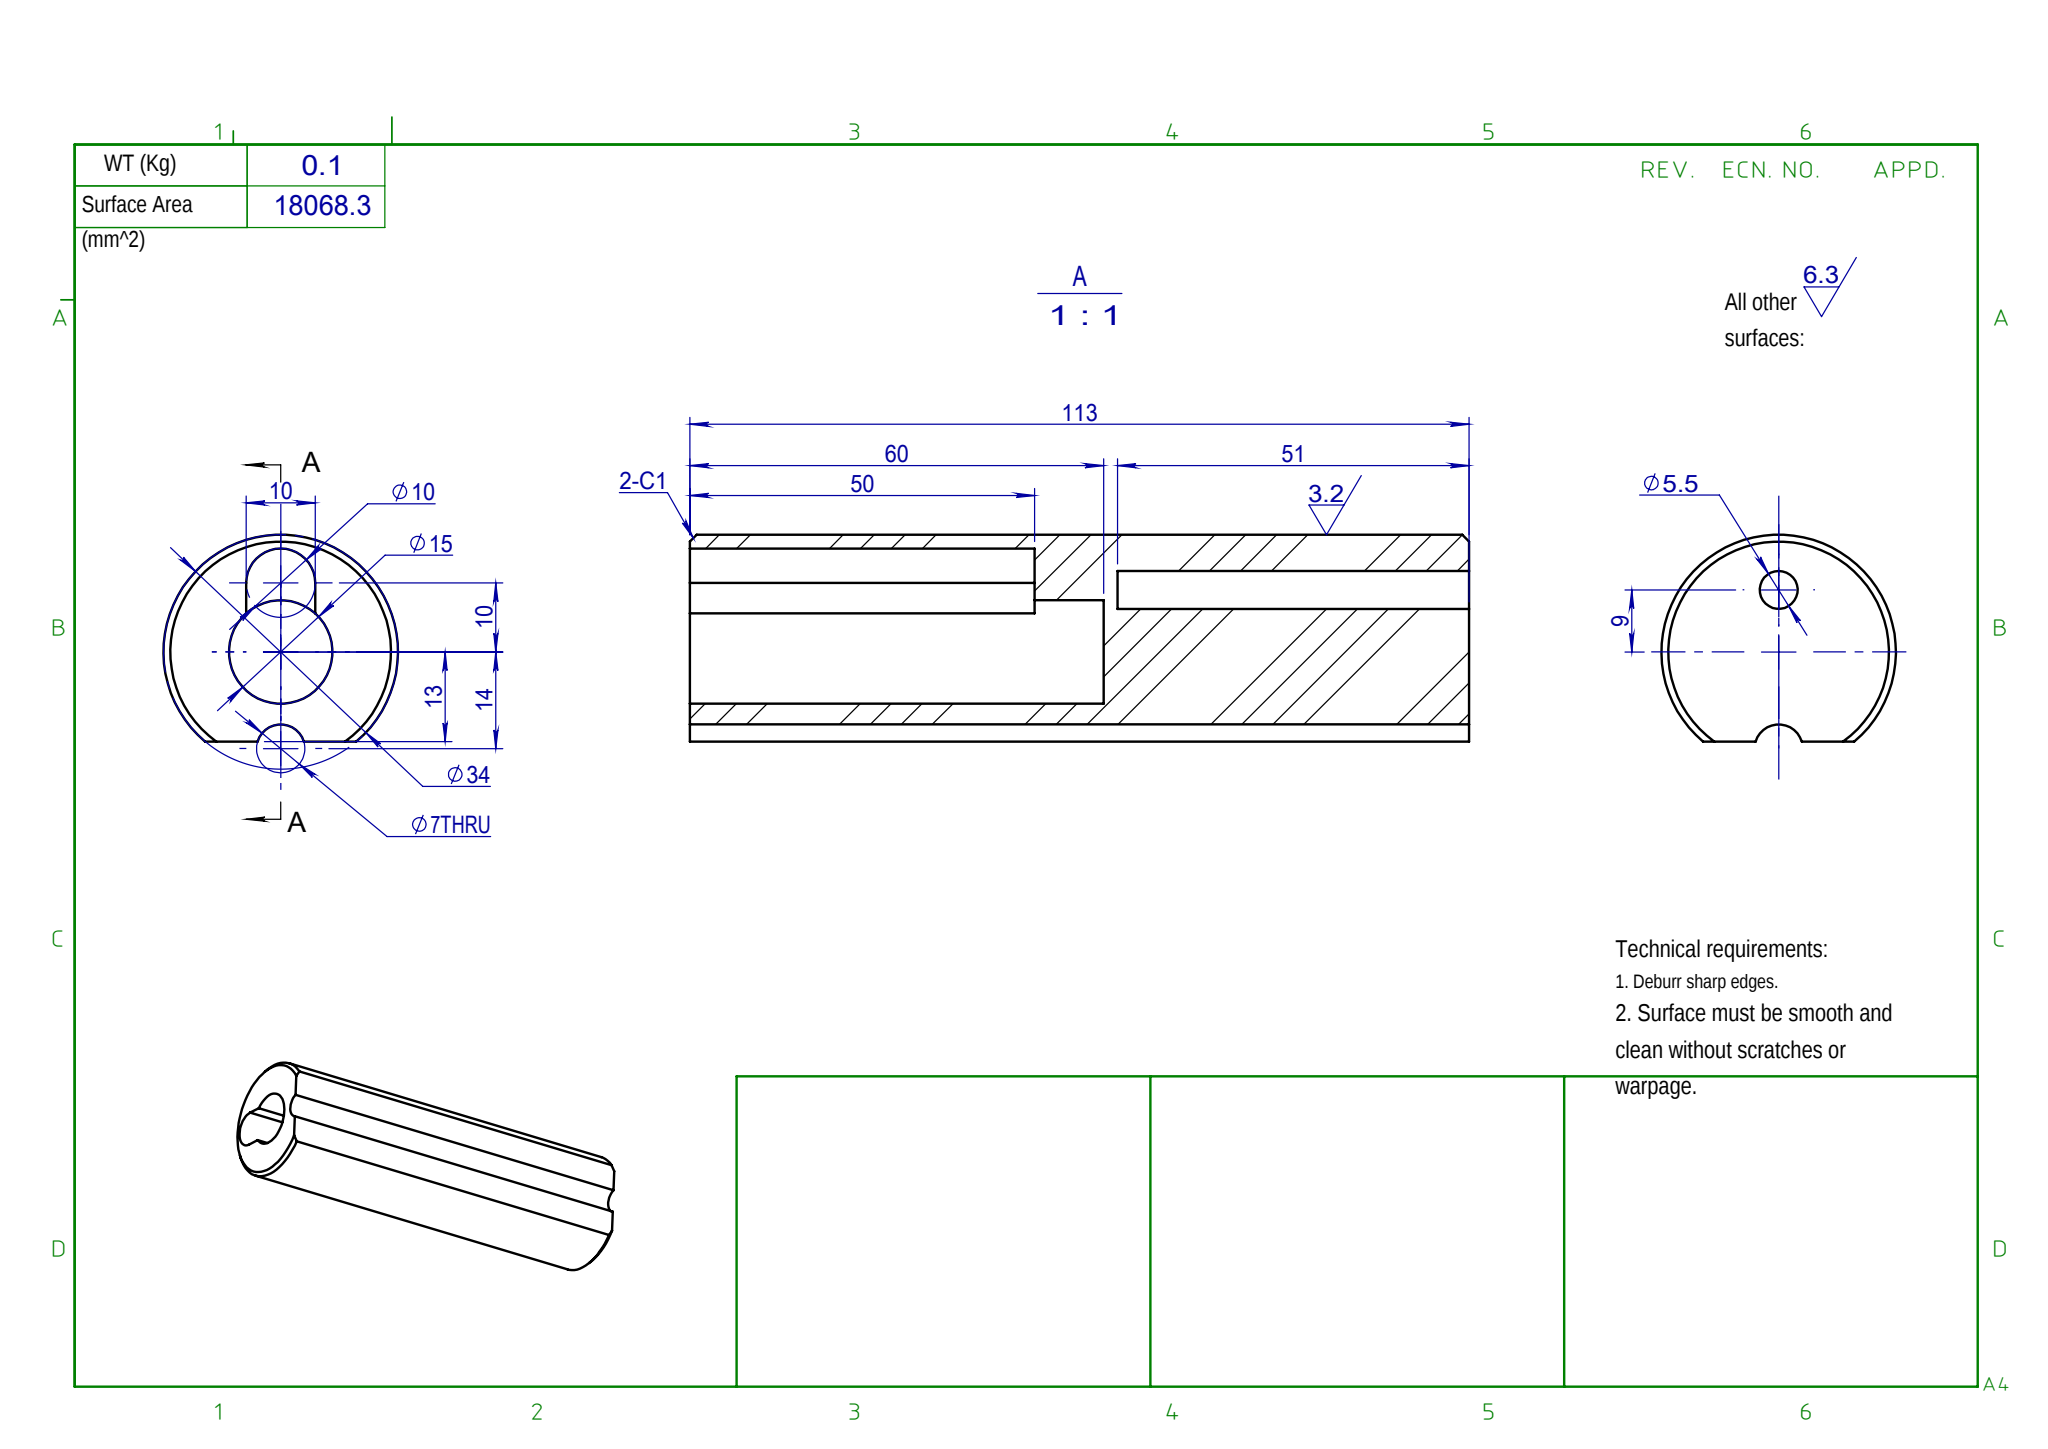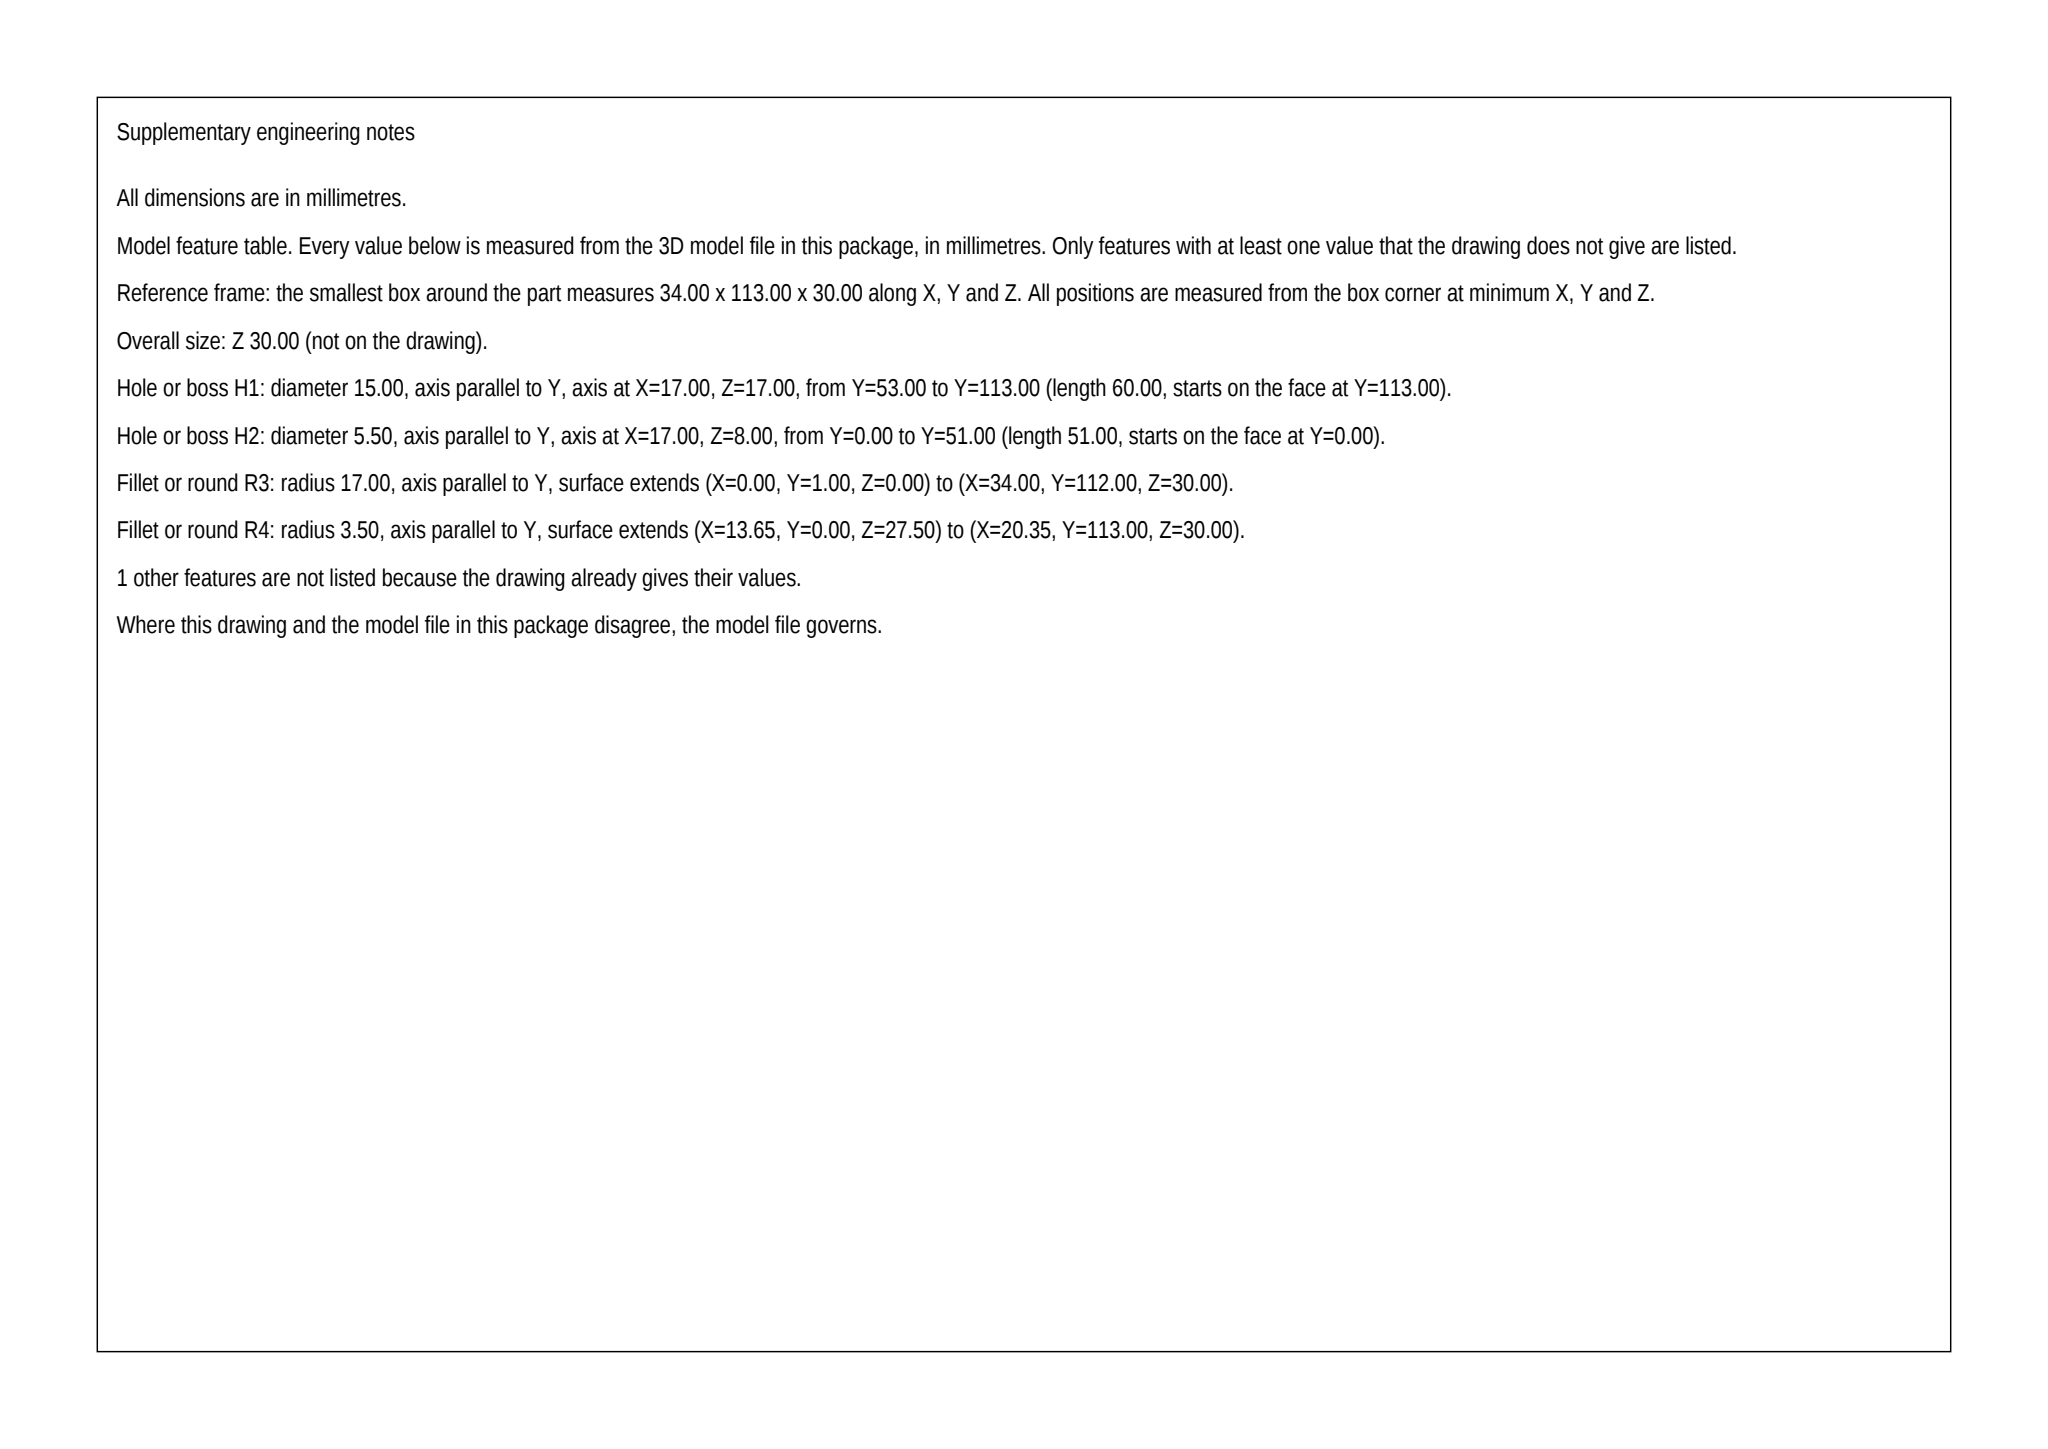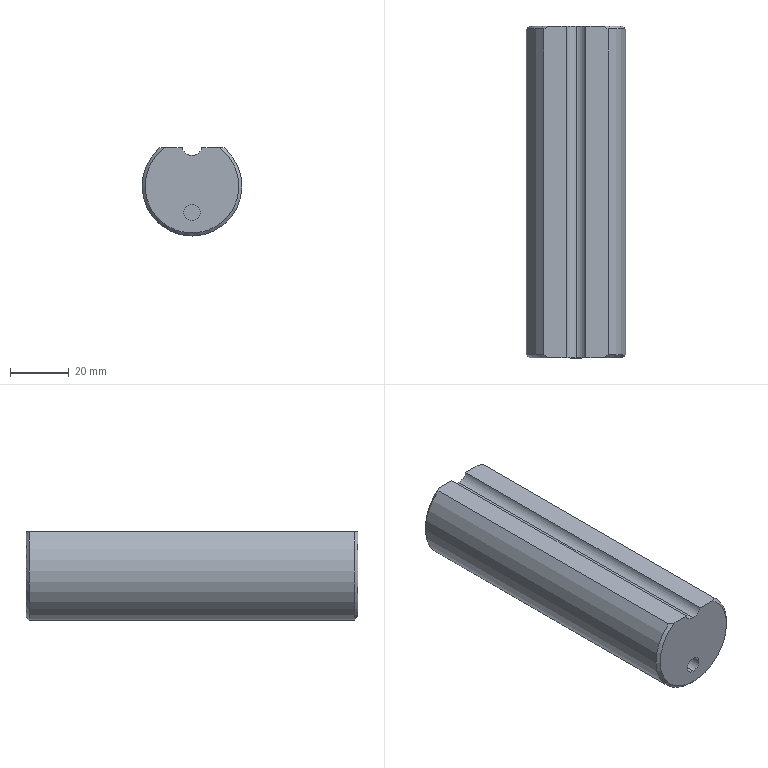Part | SolidWorks | mm | 1 solid | 21 faces | box 34 x 113 x 30 mm | volume 79016 mm3 | cylinder 9 | plane 9 | cone 3 | commonest cylinder face diameters 5.5 x2 15 x2 7 x2 34 x2 10 x1
STEP:
#1=CARTESIAN_POINT('',(0.,113.,-16.));
#2=VERTEX_POINT('',#1);
#3=CARTESIAN_POINT('',(-9.327,113.,13.));
#4=VERTEX_POINT('',#3);
#5=CARTESIAN_POINT('',(0.,113.,0.));
#6=DIRECTION('',(0.,1.,0.));
#7=DIRECTION('',(0.,0.,1.));
#8=AXIS2_PLACEMENT_3D('',#5,#6,#7);
#9=CIRCLE('',#8,16.);
#10=EDGE_CURVE('',#2,#4,#9,.T.);
#11=ORIENTED_EDGE('',*,*,#10,.F.);
#12=CARTESIAN_POINT('',(0.,112.,-17.));
#13=VERTEX_POINT('',#12);
#14=CARTESIAN_POINT('',(0.,113.,-16.));
#15=DIRECTION('',(0.,-0.7071,-0.7071));
#16=VECTOR('',#15,1000.);
#17=LINE('',#14,#16);
#18=EDGE_CURVE('',#2,#13,#17,.T.);
#19=ORIENTED_EDGE('',*,*,#18,.T.);
#20=CARTESIAN_POINT('',(-10.954,112.,13.));
#21=VERTEX_POINT('',#20);
#22=CARTESIAN_POINT('',(0.,112.,0.));
#23=DIRECTION('',(0.,-1.,0.));
#24=DIRECTION('',(0.,0.,1.));
#25=AXIS2_PLACEMENT_3D('',#22,#23,#24);
#26=CIRCLE('',#25,17.);
#27=EDGE_CURVE('',#21,#13,#26,.T.);
#28=ORIENTED_EDGE('',*,*,#27,.F.);
#29=CARTESIAN_POINT('',(-9.327,113.,13.));
#30=CARTESIAN_POINT('',(-9.878,112.679,13.));
#31=CARTESIAN_POINT('',(-10.419,112.345,13.));
#32=CARTESIAN_POINT('',(-10.954,112.,13.));
#33=B_SPLINE_CURVE_WITH_KNOTS('',3,(#29,#30,#31,#32),.UNSPECIFIED.,.F.,.F.,(4,4),(0.,0.00191),.UNSPECIFIED.);
#34=EDGE_CURVE('',#4,#21,#33,.T.);
#35=ORIENTED_EDGE('',*,*,#34,.F.);
#36=EDGE_LOOP('',(#11,#19,#28,#35));
#37=FACE_OUTER_BOUND('',#36,.T.);
#38=CARTESIAN_POINT('',(0.,113.,0.));
#39=DIRECTION('',(0.,-1.,0.));
#40=DIRECTION('',(0.,0.,-1.));
#41=AXIS2_PLACEMENT_3D('',#38,#39,#40);
#42=CONICAL_SURFACE('',#41,16.,0.7854);
#43=ADVANCED_FACE('',(#37),#42,.T.);
#44=CARTESIAN_POINT('',(0.,51.,-6.25));
#45=VERTEX_POINT('',#44);
#46=CARTESIAN_POINT('',(0.,51.,-11.75));
#47=VERTEX_POINT('',#46);
#48=CARTESIAN_POINT('',(0.,51.,-9.));
#49=DIRECTION('',(0.,-1.,0.));
#50=DIRECTION('',(0.,0.,-1.));
#51=AXIS2_PLACEMENT_3D('',#48,#49,#50);
#52=CIRCLE('',#51,2.75);
#53=EDGE_CURVE('',#45,#47,#52,.T.);
#54=ORIENTED_EDGE('',*,*,#53,.F.);
#55=CARTESIAN_POINT('',(0.,0.,-6.25));
#56=VERTEX_POINT('',#55);
#57=CARTESIAN_POINT('',(0.,51.,-6.25));
#58=DIRECTION('',(0.,-1.,0.));
#59=VECTOR('',#58,1000.);
#60=LINE('',#57,#59);
#61=EDGE_CURVE('',#45,#56,#60,.T.);
#62=ORIENTED_EDGE('',*,*,#61,.T.);
#63=CARTESIAN_POINT('',(0.,0.,-11.75));
#64=VERTEX_POINT('',#63);
#65=CARTESIAN_POINT('',(0.,0.,-9.));
#66=DIRECTION('',(0.,-1.,0.));
#67=DIRECTION('',(0.,0.,-1.));
#68=AXIS2_PLACEMENT_3D('',#65,#66,#67);
#69=CIRCLE('',#68,2.75);
#70=EDGE_CURVE('',#56,#64,#69,.T.);
#71=ORIENTED_EDGE('',*,*,#70,.T.);
#72=CARTESIAN_POINT('',(0.,51.,-11.75));
#73=DIRECTION('',(0.,-1.,0.));
#74=VECTOR('',#73,1000.);
#75=LINE('',#72,#74);
#76=EDGE_CURVE('',#47,#64,#75,.T.);
#77=ORIENTED_EDGE('',*,*,#76,.F.);
#78=EDGE_LOOP('',(#54,#62,#71,#77));
#79=FACE_OUTER_BOUND('',#78,.T.);
#80=CARTESIAN_POINT('',(0.,51.,-9.));
#81=DIRECTION('',(0.,-1.,0.));
#82=DIRECTION('',(0.,0.,-1.));
#83=AXIS2_PLACEMENT_3D('',#80,#81,#82);
#84=CYLINDRICAL_SURFACE('',#83,2.75);
#85=ADVANCED_FACE('',(#79),#84,.F.);
#86=CARTESIAN_POINT('',(0.,53.,-7.5));
#87=VERTEX_POINT('',#86);
#88=CARTESIAN_POINT('',(0.,53.,7.5));
#89=VERTEX_POINT('',#88);
#90=CARTESIAN_POINT('',(0.,53.,0.));
#91=DIRECTION('',(0.,1.,0.));
#92=DIRECTION('',(0.,0.,1.));
#93=AXIS2_PLACEMENT_3D('',#90,#91,#92);
#94=CIRCLE('',#93,7.5);
#95=EDGE_CURVE('',#87,#89,#94,.T.);
#96=ORIENTED_EDGE('',*,*,#95,.F.);
#97=CARTESIAN_POINT('',(0.,63.,-7.5));
#98=VERTEX_POINT('',#97);
#99=CARTESIAN_POINT('',(0.,53.,-7.5));
#100=DIRECTION('',(0.,1.,0.));
#101=VECTOR('',#100,1000.);
#102=LINE('',#99,#101);
#103=EDGE_CURVE('',#87,#98,#102,.T.);
#104=ORIENTED_EDGE('',*,*,#103,.T.);
#105=CARTESIAN_POINT('',(-5.,63.,-5.59));
#106=VERTEX_POINT('',#105);
#107=CARTESIAN_POINT('',(0.,63.,0.));
#108=DIRECTION('',(0.,1.,0.));
#109=DIRECTION('',(0.,0.,-1.));
#110=AXIS2_PLACEMENT_3D('',#107,#108,#109);
#111=CIRCLE('',#110,7.5);
#112=EDGE_CURVE('',#98,#106,#111,.T.);
#113=ORIENTED_EDGE('',*,*,#112,.T.);
#114=CARTESIAN_POINT('',(-5.,113.,-5.59));
#115=VERTEX_POINT('',#114);
#116=CARTESIAN_POINT('',(-5.,53.,-5.59));
#117=DIRECTION('',(0.,1.,0.));
#118=VECTOR('',#117,1000.);
#119=LINE('',#116,#118);
#120=EDGE_CURVE('',#106,#115,#119,.T.);
#121=ORIENTED_EDGE('',*,*,#120,.T.);
#122=CARTESIAN_POINT('',(0.,113.,7.5));
#123=VERTEX_POINT('',#122);
#124=CARTESIAN_POINT('',(0.,113.,0.));
#125=DIRECTION('',(0.,1.,0.));
#126=DIRECTION('',(0.,0.,1.));
#127=AXIS2_PLACEMENT_3D('',#124,#125,#126);
#128=CIRCLE('',#127,7.5);
#129=EDGE_CURVE('',#115,#123,#128,.T.);
#130=ORIENTED_EDGE('',*,*,#129,.T.);
#131=CARTESIAN_POINT('',(0.,53.,7.5));
#132=DIRECTION('',(0.,1.,0.));
#133=VECTOR('',#132,1000.);
#134=LINE('',#131,#133);
#135=EDGE_CURVE('',#89,#123,#134,.T.);
#136=ORIENTED_EDGE('',*,*,#135,.F.);
#137=EDGE_LOOP('',(#96,#104,#113,#121,#130,#136));
#138=FACE_OUTER_BOUND('',#137,.T.);
#139=CARTESIAN_POINT('',(0.,53.,0.));
#140=DIRECTION('',(0.,1.,0.));
#141=DIRECTION('',(0.,0.,1.));
#142=AXIS2_PLACEMENT_3D('',#139,#140,#141);
#143=CYLINDRICAL_SURFACE('',#142,7.5);
#144=ADVANCED_FACE('',(#138),#143,.F.);
#145=CARTESIAN_POINT('',(0.,113.,10.5));
#146=VERTEX_POINT('',#145);
#147=CARTESIAN_POINT('',(3.354,113.,13.));
#148=VERTEX_POINT('',#147);
#149=CARTESIAN_POINT('',(0.,113.,14.));
#150=DIRECTION('',(0.,-1.,0.));
#151=DIRECTION('',(0.,0.,1.));
#152=AXIS2_PLACEMENT_3D('',#149,#150,#151);
#153=CIRCLE('',#152,3.5);
#154=EDGE_CURVE('',#146,#148,#153,.T.);
#155=ORIENTED_EDGE('',*,*,#154,.F.);
#156=CARTESIAN_POINT('',(0.,0.,10.5));
#157=VERTEX_POINT('',#156);
#158=CARTESIAN_POINT('',(0.,113.,10.5));
#159=DIRECTION('',(0.,-1.,0.));
#160=VECTOR('',#159,1000.);
#161=LINE('',#158,#160);
#162=EDGE_CURVE('',#146,#157,#161,.T.);
#163=ORIENTED_EDGE('',*,*,#162,.T.);
#164=CARTESIAN_POINT('',(3.354,0.,13.));
#165=VERTEX_POINT('',#164);
#166=CARTESIAN_POINT('',(0.,0.,14.));
#167=DIRECTION('',(0.,-1.,0.));
#168=DIRECTION('',(0.,0.,1.));
#169=AXIS2_PLACEMENT_3D('',#166,#167,#168);
#170=CIRCLE('',#169,3.5);
#171=EDGE_CURVE('',#157,#165,#170,.T.);
#172=ORIENTED_EDGE('',*,*,#171,.T.);
#173=CARTESIAN_POINT('',(3.354,113.,13.));
#174=DIRECTION('',(0.,-1.,0.));
#175=VECTOR('',#174,1000.);
#176=LINE('',#173,#175);
#177=EDGE_CURVE('',#148,#165,#176,.T.);
#178=ORIENTED_EDGE('',*,*,#177,.F.);
#179=EDGE_LOOP('',(#155,#163,#172,#178));
#180=FACE_OUTER_BOUND('',#179,.T.);
#181=CARTESIAN_POINT('',(0.,113.,14.));
#182=DIRECTION('',(0.,-1.,0.));
#183=DIRECTION('',(0.,0.,-1.));
#184=AXIS2_PLACEMENT_3D('',#181,#182,#183);
#185=CYLINDRICAL_SURFACE('',#184,3.5);
#186=ADVANCED_FACE('',(#180),#185,.F.);
#187=ORIENTED_EDGE('',*,*,#27,.T.);
#188=CARTESIAN_POINT('',(0.,1.,-17.));
#189=VERTEX_POINT('',#188);
#190=CARTESIAN_POINT('',(0.,113.,-17.));
#191=DIRECTION('',(0.,-1.,0.));
#192=VECTOR('',#191,1000.);
#193=LINE('',#190,#192);
#194=EDGE_CURVE('',#13,#189,#193,.T.);
#195=ORIENTED_EDGE('',*,*,#194,.T.);
#196=CARTESIAN_POINT('',(-10.954,1.,13.));
#197=VERTEX_POINT('',#196);
#198=CARTESIAN_POINT('',(0.,1.,0.));
#199=DIRECTION('',(0.,1.,0.));
#200=DIRECTION('',(0.,0.,1.));
#201=AXIS2_PLACEMENT_3D('',#198,#199,#200);
#202=CIRCLE('',#201,17.);
#203=EDGE_CURVE('',#189,#197,#202,.T.);
#204=ORIENTED_EDGE('',*,*,#203,.T.);
#205=CARTESIAN_POINT('',(-10.954,113.,13.));
#206=DIRECTION('',(0.,-1.,0.));
#207=VECTOR('',#206,1000.);
#208=LINE('',#205,#207);
#209=EDGE_CURVE('',#21,#197,#208,.T.);
#210=ORIENTED_EDGE('',*,*,#209,.F.);
#211=EDGE_LOOP('',(#187,#195,#204,#210));
#212=FACE_OUTER_BOUND('',#211,.T.);
#213=CARTESIAN_POINT('',(0.,113.,0.));
#214=DIRECTION('',(0.,-1.,0.));
#215=DIRECTION('',(0.,0.,-1.));
#216=AXIS2_PLACEMENT_3D('',#213,#214,#215);
#217=CYLINDRICAL_SURFACE('',#216,17.);
#218=ADVANCED_FACE('',(#212),#217,.T.);
#219=CARTESIAN_POINT('',(-5.,63.,-10.));
#220=VERTEX_POINT('',#219);
#221=CARTESIAN_POINT('',(-5.,113.,-10.));
#222=VERTEX_POINT('',#221);
#223=CARTESIAN_POINT('',(-5.,63.,-10.));
#224=DIRECTION('',(0.,1.,0.));
#225=VECTOR('',#224,1000.);
#226=LINE('',#223,#225);
#227=EDGE_CURVE('',#220,#222,#226,.T.);
#228=ORIENTED_EDGE('',*,*,#227,.F.);
#229=CARTESIAN_POINT('',(5.,63.,-10.));
#230=VERTEX_POINT('',#229);
#231=CARTESIAN_POINT('',(0.,63.,-10.));
#232=DIRECTION('',(0.,1.,0.));
#233=DIRECTION('',(0.,0.,-1.));
#234=AXIS2_PLACEMENT_3D('',#231,#232,#233);
#235=CIRCLE('',#234,5.);
#236=EDGE_CURVE('',#230,#220,#235,.T.);
#237=ORIENTED_EDGE('',*,*,#236,.F.);
#238=CARTESIAN_POINT('',(5.,113.,-10.));
#239=VERTEX_POINT('',#238);
#240=CARTESIAN_POINT('',(5.,63.,-10.));
#241=DIRECTION('',(0.,-1.,0.));
#242=VECTOR('',#241,1000.);
#243=LINE('',#240,#242);
#244=EDGE_CURVE('',#239,#230,#243,.T.);
#245=ORIENTED_EDGE('',*,*,#244,.F.);
#246=CARTESIAN_POINT('',(0.,113.,-10.));
#247=DIRECTION('',(0.,1.,0.));
#248=DIRECTION('',(0.,0.,1.));
#249=AXIS2_PLACEMENT_3D('',#246,#247,#248);
#250=CIRCLE('',#249,5.);
#251=EDGE_CURVE('',#239,#222,#250,.T.);
#252=ORIENTED_EDGE('',*,*,#251,.T.);
#253=EDGE_LOOP('',(#228,#237,#245,#252));
#254=FACE_OUTER_BOUND('',#253,.T.);
#255=CARTESIAN_POINT('',(0.,63.,-10.));
#256=DIRECTION('',(0.,1.,0.));
#257=DIRECTION('',(0.,0.,1.));
#258=AXIS2_PLACEMENT_3D('',#255,#256,#257);
#259=CYLINDRICAL_SURFACE('',#258,5.);
#260=ADVANCED_FACE('',(#254),#259,.F.);
#261=ORIENTED_EDGE('',*,*,#194,.F.);
#262=CARTESIAN_POINT('',(10.954,112.,13.));
#263=VERTEX_POINT('',#262);
#264=CARTESIAN_POINT('',(0.,112.,0.));
#265=DIRECTION('',(0.,-1.,0.));
#266=DIRECTION('',(0.,0.,1.));
#267=AXIS2_PLACEMENT_3D('',#264,#265,#266);
#268=CIRCLE('',#267,17.);
#269=EDGE_CURVE('',#13,#263,#268,.T.);
#270=ORIENTED_EDGE('',*,*,#269,.T.);
#271=CARTESIAN_POINT('',(10.954,1.,13.));
#272=VERTEX_POINT('',#271);
#273=CARTESIAN_POINT('',(10.954,113.,13.));
#274=DIRECTION('',(0.,-1.,0.));
#275=VECTOR('',#274,1000.);
#276=LINE('',#273,#275);
#277=EDGE_CURVE('',#263,#272,#276,.T.);
#278=ORIENTED_EDGE('',*,*,#277,.T.);
#279=CARTESIAN_POINT('',(0.,1.,0.));
#280=DIRECTION('',(0.,1.,0.));
#281=DIRECTION('',(0.,0.,1.));
#282=AXIS2_PLACEMENT_3D('',#279,#280,#281);
#283=CIRCLE('',#282,17.);
#284=EDGE_CURVE('',#272,#189,#283,.T.);
#285=ORIENTED_EDGE('',*,*,#284,.T.);
#286=EDGE_LOOP('',(#261,#270,#278,#285));
#287=FACE_OUTER_BOUND('',#286,.T.);
#288=CARTESIAN_POINT('',(0.,113.,0.));
#289=DIRECTION('',(0.,-1.,0.));
#290=DIRECTION('',(0.,0.,-1.));
#291=AXIS2_PLACEMENT_3D('',#288,#289,#290);
#292=CYLINDRICAL_SURFACE('',#291,17.);
#293=ADVANCED_FACE('',(#287),#292,.T.);
#294=CARTESIAN_POINT('',(-3.354,113.,13.));
#295=VERTEX_POINT('',#294);
#296=CARTESIAN_POINT('',(-10.954,113.,13.));
#297=DIRECTION('',(1.,0.,-0.));
#298=VECTOR('',#297,1000.);
#299=LINE('',#296,#298);
#300=EDGE_CURVE('',#4,#295,#299,.T.);
#301=ORIENTED_EDGE('',*,*,#300,.F.);
#302=ORIENTED_EDGE('',*,*,#34,.T.);
#303=ORIENTED_EDGE('',*,*,#209,.T.);
#304=CARTESIAN_POINT('',(-9.327,0.,13.));
#305=VERTEX_POINT('',#304);
#306=CARTESIAN_POINT('',(-10.954,1.,13.));
#307=CARTESIAN_POINT('',(-10.419,0.6551,13.));
#308=CARTESIAN_POINT('',(-9.878,0.3207,13.));
#309=CARTESIAN_POINT('',(-9.327,0.,13.));
#310=B_SPLINE_CURVE_WITH_KNOTS('',3,(#306,#307,#308,#309),.UNSPECIFIED.,.F.,.F.,(4,4),(0.,0.00191),.UNSPECIFIED.);
#311=EDGE_CURVE('',#197,#305,#310,.T.);
#312=ORIENTED_EDGE('',*,*,#311,.T.);
#313=CARTESIAN_POINT('',(-3.354,0.,13.));
#314=VERTEX_POINT('',#313);
#315=CARTESIAN_POINT('',(-10.954,0.,13.));
#316=DIRECTION('',(1.,0.,-0.));
#317=VECTOR('',#316,1000.);
#318=LINE('',#315,#317);
#319=EDGE_CURVE('',#305,#314,#318,.T.);
#320=ORIENTED_EDGE('',*,*,#319,.T.);
#321=CARTESIAN_POINT('',(-3.354,113.,13.));
#322=DIRECTION('',(0.,-1.,0.));
#323=VECTOR('',#322,1000.);
#324=LINE('',#321,#323);
#325=EDGE_CURVE('',#295,#314,#324,.T.);
#326=ORIENTED_EDGE('',*,*,#325,.F.);
#327=EDGE_LOOP('',(#301,#302,#303,#312,#320,#326));
#328=FACE_OUTER_BOUND('',#327,.T.);
#329=CARTESIAN_POINT('',(-10.954,113.,13.));
#330=DIRECTION('',(-0.,0.,-1.));
#331=DIRECTION('',(-1.,0.,0.));
#332=AXIS2_PLACEMENT_3D('',#329,#330,#331);
#333=PLANE('',#332);
#334=ADVANCED_FACE('',(#328),#333,.F.);
#335=ORIENTED_EDGE('',*,*,#162,.F.);
#336=CARTESIAN_POINT('',(0.,113.,14.));
#337=DIRECTION('',(0.,-1.,0.));
#338=DIRECTION('',(0.,0.,1.));
#339=AXIS2_PLACEMENT_3D('',#336,#337,#338);
#340=CIRCLE('',#339,3.5);
#341=EDGE_CURVE('',#295,#146,#340,.T.);
#342=ORIENTED_EDGE('',*,*,#341,.F.);
#343=ORIENTED_EDGE('',*,*,#325,.T.);
#344=CARTESIAN_POINT('',(0.,0.,14.));
#345=DIRECTION('',(0.,-1.,0.));
#346=DIRECTION('',(0.,0.,1.));
#347=AXIS2_PLACEMENT_3D('',#344,#345,#346);
#348=CIRCLE('',#347,3.5);
#349=EDGE_CURVE('',#314,#157,#348,.T.);
#350=ORIENTED_EDGE('',*,*,#349,.T.);
#351=EDGE_LOOP('',(#335,#342,#343,#350));
#352=FACE_OUTER_BOUND('',#351,.T.);
#353=CARTESIAN_POINT('',(0.,113.,14.));
#354=DIRECTION('',(0.,-1.,0.));
#355=DIRECTION('',(0.,0.,-1.));
#356=AXIS2_PLACEMENT_3D('',#353,#354,#355);
#357=CYLINDRICAL_SURFACE('',#356,3.5);
#358=ADVANCED_FACE('',(#352),#357,.F.);
#359=ORIENTED_EDGE('',*,*,#277,.F.);
#360=CARTESIAN_POINT('',(9.327,113.,13.));
#361=VERTEX_POINT('',#360);
#362=CARTESIAN_POINT('',(10.954,112.,13.));
#363=CARTESIAN_POINT('',(10.419,112.345,13.));
#364=CARTESIAN_POINT('',(9.878,112.679,13.));
#365=CARTESIAN_POINT('',(9.327,113.,13.));
#366=B_SPLINE_CURVE_WITH_KNOTS('',3,(#362,#363,#364,#365),.UNSPECIFIED.,.F.,.F.,(4,4),(0.,0.00191),.UNSPECIFIED.);
#367=EDGE_CURVE('',#263,#361,#366,.T.);
#368=ORIENTED_EDGE('',*,*,#367,.T.);
#369=CARTESIAN_POINT('',(3.354,113.,13.));
#370=DIRECTION('',(1.,0.,-0.));
#371=VECTOR('',#370,1000.);
#372=LINE('',#369,#371);
#373=EDGE_CURVE('',#148,#361,#372,.T.);
#374=ORIENTED_EDGE('',*,*,#373,.F.);
#375=ORIENTED_EDGE('',*,*,#177,.T.);
#376=CARTESIAN_POINT('',(9.327,0.,13.));
#377=VERTEX_POINT('',#376);
#378=CARTESIAN_POINT('',(3.354,0.,13.));
#379=DIRECTION('',(1.,0.,-0.));
#380=VECTOR('',#379,1000.);
#381=LINE('',#378,#380);
#382=EDGE_CURVE('',#165,#377,#381,.T.);
#383=ORIENTED_EDGE('',*,*,#382,.T.);
#384=CARTESIAN_POINT('',(9.327,0.,13.));
#385=CARTESIAN_POINT('',(9.878,0.3207,13.));
#386=CARTESIAN_POINT('',(10.419,0.6551,13.));
#387=CARTESIAN_POINT('',(10.954,1.,13.));
#388=B_SPLINE_CURVE_WITH_KNOTS('',3,(#384,#385,#386,#387),.UNSPECIFIED.,.F.,.F.,(4,4),(0.,0.00191),.UNSPECIFIED.);
#389=EDGE_CURVE('',#377,#272,#388,.T.);
#390=ORIENTED_EDGE('',*,*,#389,.T.);
#391=EDGE_LOOP('',(#359,#368,#374,#375,#383,#390));
#392=FACE_OUTER_BOUND('',#391,.T.);
#393=CARTESIAN_POINT('',(3.354,113.,13.));
#394=DIRECTION('',(-0.,0.,-1.));
#395=DIRECTION('',(-1.,0.,0.));
#396=AXIS2_PLACEMENT_3D('',#393,#394,#395);
#397=PLANE('',#396);
#398=ADVANCED_FACE('',(#392),#397,.F.);
#399=CARTESIAN_POINT('',(-5.,113.,-4.));
#400=DIRECTION('',(0.,0.,1.));
#401=VECTOR('',#400,1000.);
#402=LINE('',#399,#401);
#403=EDGE_CURVE('',#222,#115,#402,.T.);
#404=ORIENTED_EDGE('',*,*,#403,.F.);
#405=ORIENTED_EDGE('',*,*,#251,.F.);
#406=CARTESIAN_POINT('',(5.,113.,-5.59));
#407=VERTEX_POINT('',#406);
#408=CARTESIAN_POINT('',(5.,113.,-4.));
#409=DIRECTION('',(0.,0.,-1.));
#410=VECTOR('',#409,1000.);
#411=LINE('',#408,#410);
#412=EDGE_CURVE('',#407,#239,#411,.T.);
#413=ORIENTED_EDGE('',*,*,#412,.F.);
#414=CARTESIAN_POINT('',(0.,113.,0.));
#415=DIRECTION('',(0.,1.,0.));
#416=DIRECTION('',(0.,0.,1.));
#417=AXIS2_PLACEMENT_3D('',#414,#415,#416);
#418=CIRCLE('',#417,7.5);
#419=EDGE_CURVE('',#123,#407,#418,.T.);
#420=ORIENTED_EDGE('',*,*,#419,.F.);
#421=ORIENTED_EDGE('',*,*,#129,.F.);
#422=EDGE_LOOP('',(#404,#405,#413,#420,#421));
#423=FACE_BOUND('',#422,.T.);
#424=ORIENTED_EDGE('',*,*,#373,.T.);
#425=CARTESIAN_POINT('',(0.,113.,0.));
#426=DIRECTION('',(0.,1.,0.));
#427=DIRECTION('',(0.,0.,1.));
#428=AXIS2_PLACEMENT_3D('',#425,#426,#427);
#429=CIRCLE('',#428,16.);
#430=EDGE_CURVE('',#361,#2,#429,.T.);
#431=ORIENTED_EDGE('',*,*,#430,.T.);
#432=ORIENTED_EDGE('',*,*,#10,.T.);
#433=ORIENTED_EDGE('',*,*,#300,.T.);
#434=ORIENTED_EDGE('',*,*,#341,.T.);
#435=ORIENTED_EDGE('',*,*,#154,.T.);
#436=EDGE_LOOP('',(#424,#431,#432,#433,#434,#435));
#437=FACE_OUTER_BOUND('',#436,.T.);
#438=CARTESIAN_POINT('',(0.,113.,0.));
#439=DIRECTION('',(0.,1.,0.));
#440=DIRECTION('',(0.,0.,1.));
#441=AXIS2_PLACEMENT_3D('',#438,#439,#440);
#442=PLANE('',#441);
#443=ADVANCED_FACE('',(#423,#437),#442,.T.);
#444=CARTESIAN_POINT('',(0.,0.,-9.));
#445=DIRECTION('',(0.,-1.,0.));
#446=DIRECTION('',(0.,0.,-1.));
#447=AXIS2_PLACEMENT_3D('',#444,#445,#446);
#448=CIRCLE('',#447,2.75);
#449=EDGE_CURVE('',#64,#56,#448,.T.);
#450=ORIENTED_EDGE('',*,*,#449,.F.);
#451=ORIENTED_EDGE('',*,*,#70,.F.);
#452=EDGE_LOOP('',(#450,#451));
#453=FACE_BOUND('',#452,.T.);
#454=ORIENTED_EDGE('',*,*,#319,.F.);
#455=CARTESIAN_POINT('',(0.,0.,0.));
#456=DIRECTION('',(0.,-1.,0.));
#457=DIRECTION('',(0.,0.,1.));
#458=AXIS2_PLACEMENT_3D('',#455,#456,#457);
#459=CIRCLE('',#458,16.);
#460=EDGE_CURVE('',#305,#377,#459,.T.);
#461=ORIENTED_EDGE('',*,*,#460,.T.);
#462=ORIENTED_EDGE('',*,*,#382,.F.);
#463=ORIENTED_EDGE('',*,*,#171,.F.);
#464=ORIENTED_EDGE('',*,*,#349,.F.);
#465=EDGE_LOOP('',(#454,#461,#462,#463,#464));
#466=FACE_OUTER_BOUND('',#465,.T.);
#467=CARTESIAN_POINT('',(0.,0.,0.));
#468=DIRECTION('',(0.,1.,0.));
#469=DIRECTION('',(0.,0.,1.));
#470=AXIS2_PLACEMENT_3D('',#467,#468,#469);
#471=PLANE('',#470);
#472=ADVANCED_FACE('',(#453,#466),#471,.F.);
#473=ORIENTED_EDGE('',*,*,#103,.F.);
#474=CARTESIAN_POINT('',(0.,53.,0.));
#475=DIRECTION('',(0.,1.,0.));
#476=DIRECTION('',(0.,0.,1.));
#477=AXIS2_PLACEMENT_3D('',#474,#475,#476);
#478=CIRCLE('',#477,7.5);
#479=EDGE_CURVE('',#89,#87,#478,.T.);
#480=ORIENTED_EDGE('',*,*,#479,.F.);
#481=ORIENTED_EDGE('',*,*,#135,.T.);
#482=ORIENTED_EDGE('',*,*,#419,.T.);
#483=CARTESIAN_POINT('',(5.,63.,-5.59));
#484=VERTEX_POINT('',#483);
#485=CARTESIAN_POINT('',(5.,53.,-5.59));
#486=DIRECTION('',(0.,-1.,0.));
#487=VECTOR('',#486,1000.);
#488=LINE('',#485,#487);
#489=EDGE_CURVE('',#407,#484,#488,.T.);
#490=ORIENTED_EDGE('',*,*,#489,.T.);
#491=CARTESIAN_POINT('',(0.,63.,0.));
#492=DIRECTION('',(0.,1.,0.));
#493=DIRECTION('',(-0.,0.,-1.));
#494=AXIS2_PLACEMENT_3D('',#491,#492,#493);
#495=CIRCLE('',#494,7.5);
#496=EDGE_CURVE('',#484,#98,#495,.T.);
#497=ORIENTED_EDGE('',*,*,#496,.T.);
#498=EDGE_LOOP('',(#473,#480,#481,#482,#490,#497));
#499=FACE_OUTER_BOUND('',#498,.T.);
#500=CARTESIAN_POINT('',(0.,53.,0.));
#501=DIRECTION('',(0.,1.,0.));
#502=DIRECTION('',(0.,0.,1.));
#503=AXIS2_PLACEMENT_3D('',#500,#501,#502);
#504=CYLINDRICAL_SURFACE('',#503,7.5);
#505=ADVANCED_FACE('',(#499),#504,.F.);
#506=ORIENTED_EDGE('',*,*,#479,.T.);
#507=ORIENTED_EDGE('',*,*,#95,.T.);
#508=EDGE_LOOP('',(#506,#507));
#509=FACE_OUTER_BOUND('',#508,.T.);
#510=CARTESIAN_POINT('',(0.,53.,0.));
#511=DIRECTION('',(0.,1.,0.));
#512=DIRECTION('',(0.,0.,1.));
#513=AXIS2_PLACEMENT_3D('',#510,#511,#512);
#514=PLANE('',#513);
#515=ADVANCED_FACE('',(#509),#514,.T.);
#516=ORIENTED_EDGE('',*,*,#61,.F.);
#517=CARTESIAN_POINT('',(0.,51.,-9.));
#518=DIRECTION('',(0.,-1.,0.));
#519=DIRECTION('',(0.,0.,-1.));
#520=AXIS2_PLACEMENT_3D('',#517,#518,#519);
#521=CIRCLE('',#520,2.75);
#522=EDGE_CURVE('',#47,#45,#521,.T.);
#523=ORIENTED_EDGE('',*,*,#522,.F.);
#524=ORIENTED_EDGE('',*,*,#76,.T.);
#525=ORIENTED_EDGE('',*,*,#449,.T.);
#526=EDGE_LOOP('',(#516,#523,#524,#525));
#527=FACE_OUTER_BOUND('',#526,.T.);
#528=CARTESIAN_POINT('',(0.,51.,-9.));
#529=DIRECTION('',(0.,-1.,0.));
#530=DIRECTION('',(0.,0.,-1.));
#531=AXIS2_PLACEMENT_3D('',#528,#529,#530);
#532=CYLINDRICAL_SURFACE('',#531,2.75);
#533=ADVANCED_FACE('',(#527),#532,.F.);
#534=ORIENTED_EDGE('',*,*,#522,.T.);
#535=ORIENTED_EDGE('',*,*,#53,.T.);
#536=EDGE_LOOP('',(#534,#535));
#537=FACE_OUTER_BOUND('',#536,.T.);
#538=CARTESIAN_POINT('',(0.,51.,-9.));
#539=DIRECTION('',(0.,-1.,0.));
#540=DIRECTION('',(0.,0.,-1.));
#541=AXIS2_PLACEMENT_3D('',#538,#539,#540);
#542=PLANE('',#541);
#543=ADVANCED_FACE('',(#537),#542,.T.);
#544=CARTESIAN_POINT('',(-5.,63.,-4.));
#545=DIRECTION('',(0.,0.,1.));
#546=VECTOR('',#545,1000.);
#547=LINE('',#544,#546);
#548=EDGE_CURVE('',#220,#106,#547,.T.);
#549=ORIENTED_EDGE('',*,*,#548,.F.);
#550=ORIENTED_EDGE('',*,*,#227,.T.);
#551=ORIENTED_EDGE('',*,*,#403,.T.);
#552=ORIENTED_EDGE('',*,*,#120,.F.);
#553=EDGE_LOOP('',(#549,#550,#551,#552));
#554=FACE_OUTER_BOUND('',#553,.T.);
#555=CARTESIAN_POINT('',(-5.,63.,-4.));
#556=DIRECTION('',(-1.,0.,0.));
#557=DIRECTION('',(0.,0.,1.));
#558=AXIS2_PLACEMENT_3D('',#555,#556,#557);
#559=PLANE('',#558);
#560=ADVANCED_FACE('',(#554),#559,.F.);
#561=ORIENTED_EDGE('',*,*,#412,.T.);
#562=ORIENTED_EDGE('',*,*,#244,.T.);
#563=CARTESIAN_POINT('',(5.,63.,-4.));
#564=DIRECTION('',(0.,0.,-1.));
#565=VECTOR('',#564,1000.);
#566=LINE('',#563,#565);
#567=EDGE_CURVE('',#484,#230,#566,.T.);
#568=ORIENTED_EDGE('',*,*,#567,.F.);
#569=ORIENTED_EDGE('',*,*,#489,.F.);
#570=EDGE_LOOP('',(#561,#562,#568,#569));
#571=FACE_OUTER_BOUND('',#570,.T.);
#572=CARTESIAN_POINT('',(5.,63.,-4.));
#573=DIRECTION('',(1.,0.,0.));
#574=DIRECTION('',(0.,0.,-1.));
#575=AXIS2_PLACEMENT_3D('',#572,#573,#574);
#576=PLANE('',#575);
#577=ADVANCED_FACE('',(#571),#576,.F.);
#578=ORIENTED_EDGE('',*,*,#567,.T.);
#579=ORIENTED_EDGE('',*,*,#236,.T.);
#580=ORIENTED_EDGE('',*,*,#548,.T.);
#581=ORIENTED_EDGE('',*,*,#112,.F.);
#582=ORIENTED_EDGE('',*,*,#496,.F.);
#583=EDGE_LOOP('',(#578,#579,#580,#581,#582));
#584=FACE_OUTER_BOUND('',#583,.T.);
#585=CARTESIAN_POINT('',(-5.,63.,-15.));
#586=DIRECTION('',(0.,-1.,0.));
#587=DIRECTION('',(0.,0.,-1.));
#588=AXIS2_PLACEMENT_3D('',#585,#586,#587);
#589=PLANE('',#588);
#590=ADVANCED_FACE('',(#584),#589,.F.);
#591=ORIENTED_EDGE('',*,*,#18,.F.);
#592=ORIENTED_EDGE('',*,*,#430,.F.);
#593=ORIENTED_EDGE('',*,*,#367,.F.);
#594=ORIENTED_EDGE('',*,*,#269,.F.);
#595=EDGE_LOOP('',(#591,#592,#593,#594));
#596=FACE_OUTER_BOUND('',#595,.T.);
#597=CARTESIAN_POINT('',(0.,113.,0.));
#598=DIRECTION('',(0.,-1.,0.));
#599=DIRECTION('',(0.,0.,-1.));
#600=AXIS2_PLACEMENT_3D('',#597,#598,#599);
#601=CONICAL_SURFACE('',#600,16.,0.7854);
#602=ADVANCED_FACE('',(#596),#601,.T.);
#603=ORIENTED_EDGE('',*,*,#389,.F.);
#604=ORIENTED_EDGE('',*,*,#460,.F.);
#605=ORIENTED_EDGE('',*,*,#311,.F.);
#606=ORIENTED_EDGE('',*,*,#203,.F.);
#607=ORIENTED_EDGE('',*,*,#284,.F.);
#608=EDGE_LOOP('',(#603,#604,#605,#606,#607));
#609=FACE_OUTER_BOUND('',#608,.T.);
#610=CARTESIAN_POINT('',(0.,1.,0.));
#611=DIRECTION('',(0.,1.,0.));
#612=DIRECTION('',(0.,0.,1.));
#613=AXIS2_PLACEMENT_3D('',#610,#611,#612);
#614=CONICAL_SURFACE('',#613,17.,0.7854);
#615=ADVANCED_FACE('',(#609),#614,.T.);
#616=CLOSED_SHELL('',(#43,#85,#144,#186,#218,#260,#293,#334,#358,#398,#443,#472,#505,#515,#533,#543,#560,#577,#590,#602,#615));
#617=MANIFOLD_SOLID_BREP('',#616);
#618=CARTESIAN_POINT('',(0.,0.,0.));
#619=DIRECTION('',(0.,0.,1.));
#620=DIRECTION('',(1.,0.,0.));
#621=AXIS2_PLACEMENT_3D('',#618,#619,#620);
#622=(LENGTH_UNIT()NAMED_UNIT(*)SI_UNIT(.MILLI.,.METRE.));
#623=UNCERTAINTY_MEASURE_WITH_UNIT(LENGTH_MEASURE(0.00001),#622,'','');
#624=(NAMED_UNIT(*)PLANE_ANGLE_UNIT()SI_UNIT($,.RADIAN.));
#625=(NAMED_UNIT(*)SI_UNIT($,.STERADIAN.)SOLID_ANGLE_UNIT());
#626=(GEOMETRIC_REPRESENTATION_CONTEXT(3)GLOBAL_UNCERTAINTY_ASSIGNED_CONTEXT((#623))GLOBAL_UNIT_ASSIGNED_CONTEXT((#622,#624,#625))REPRESENTATION_CONTEXT('',''));
#627=ADVANCED_BREP_SHAPE_REPRESENTATION('',(#617,#621),#626);